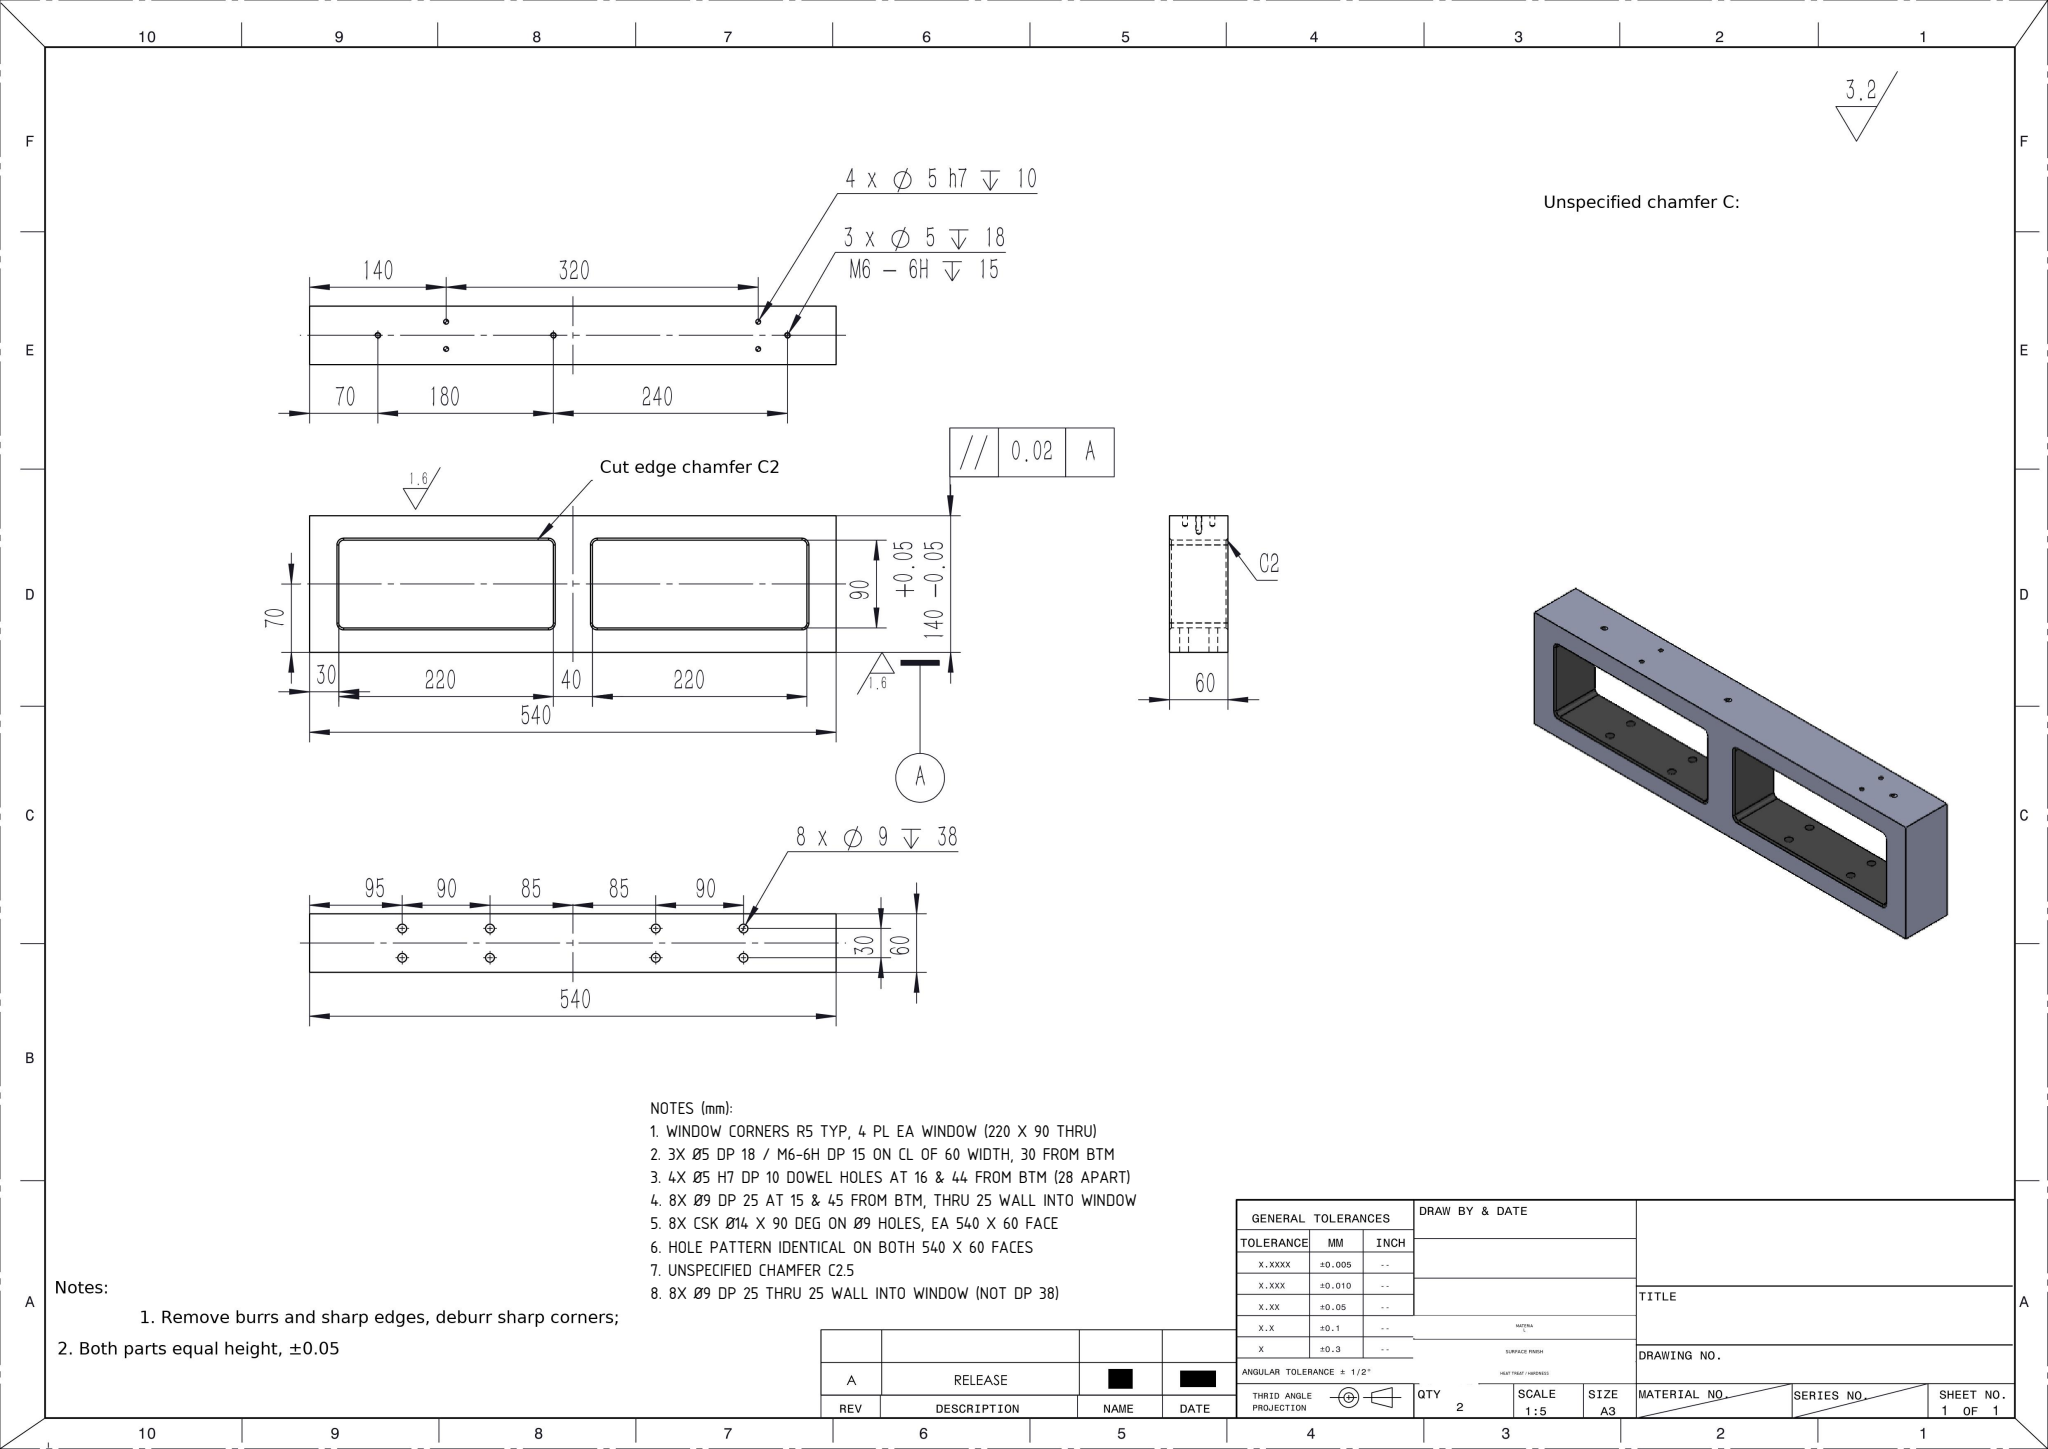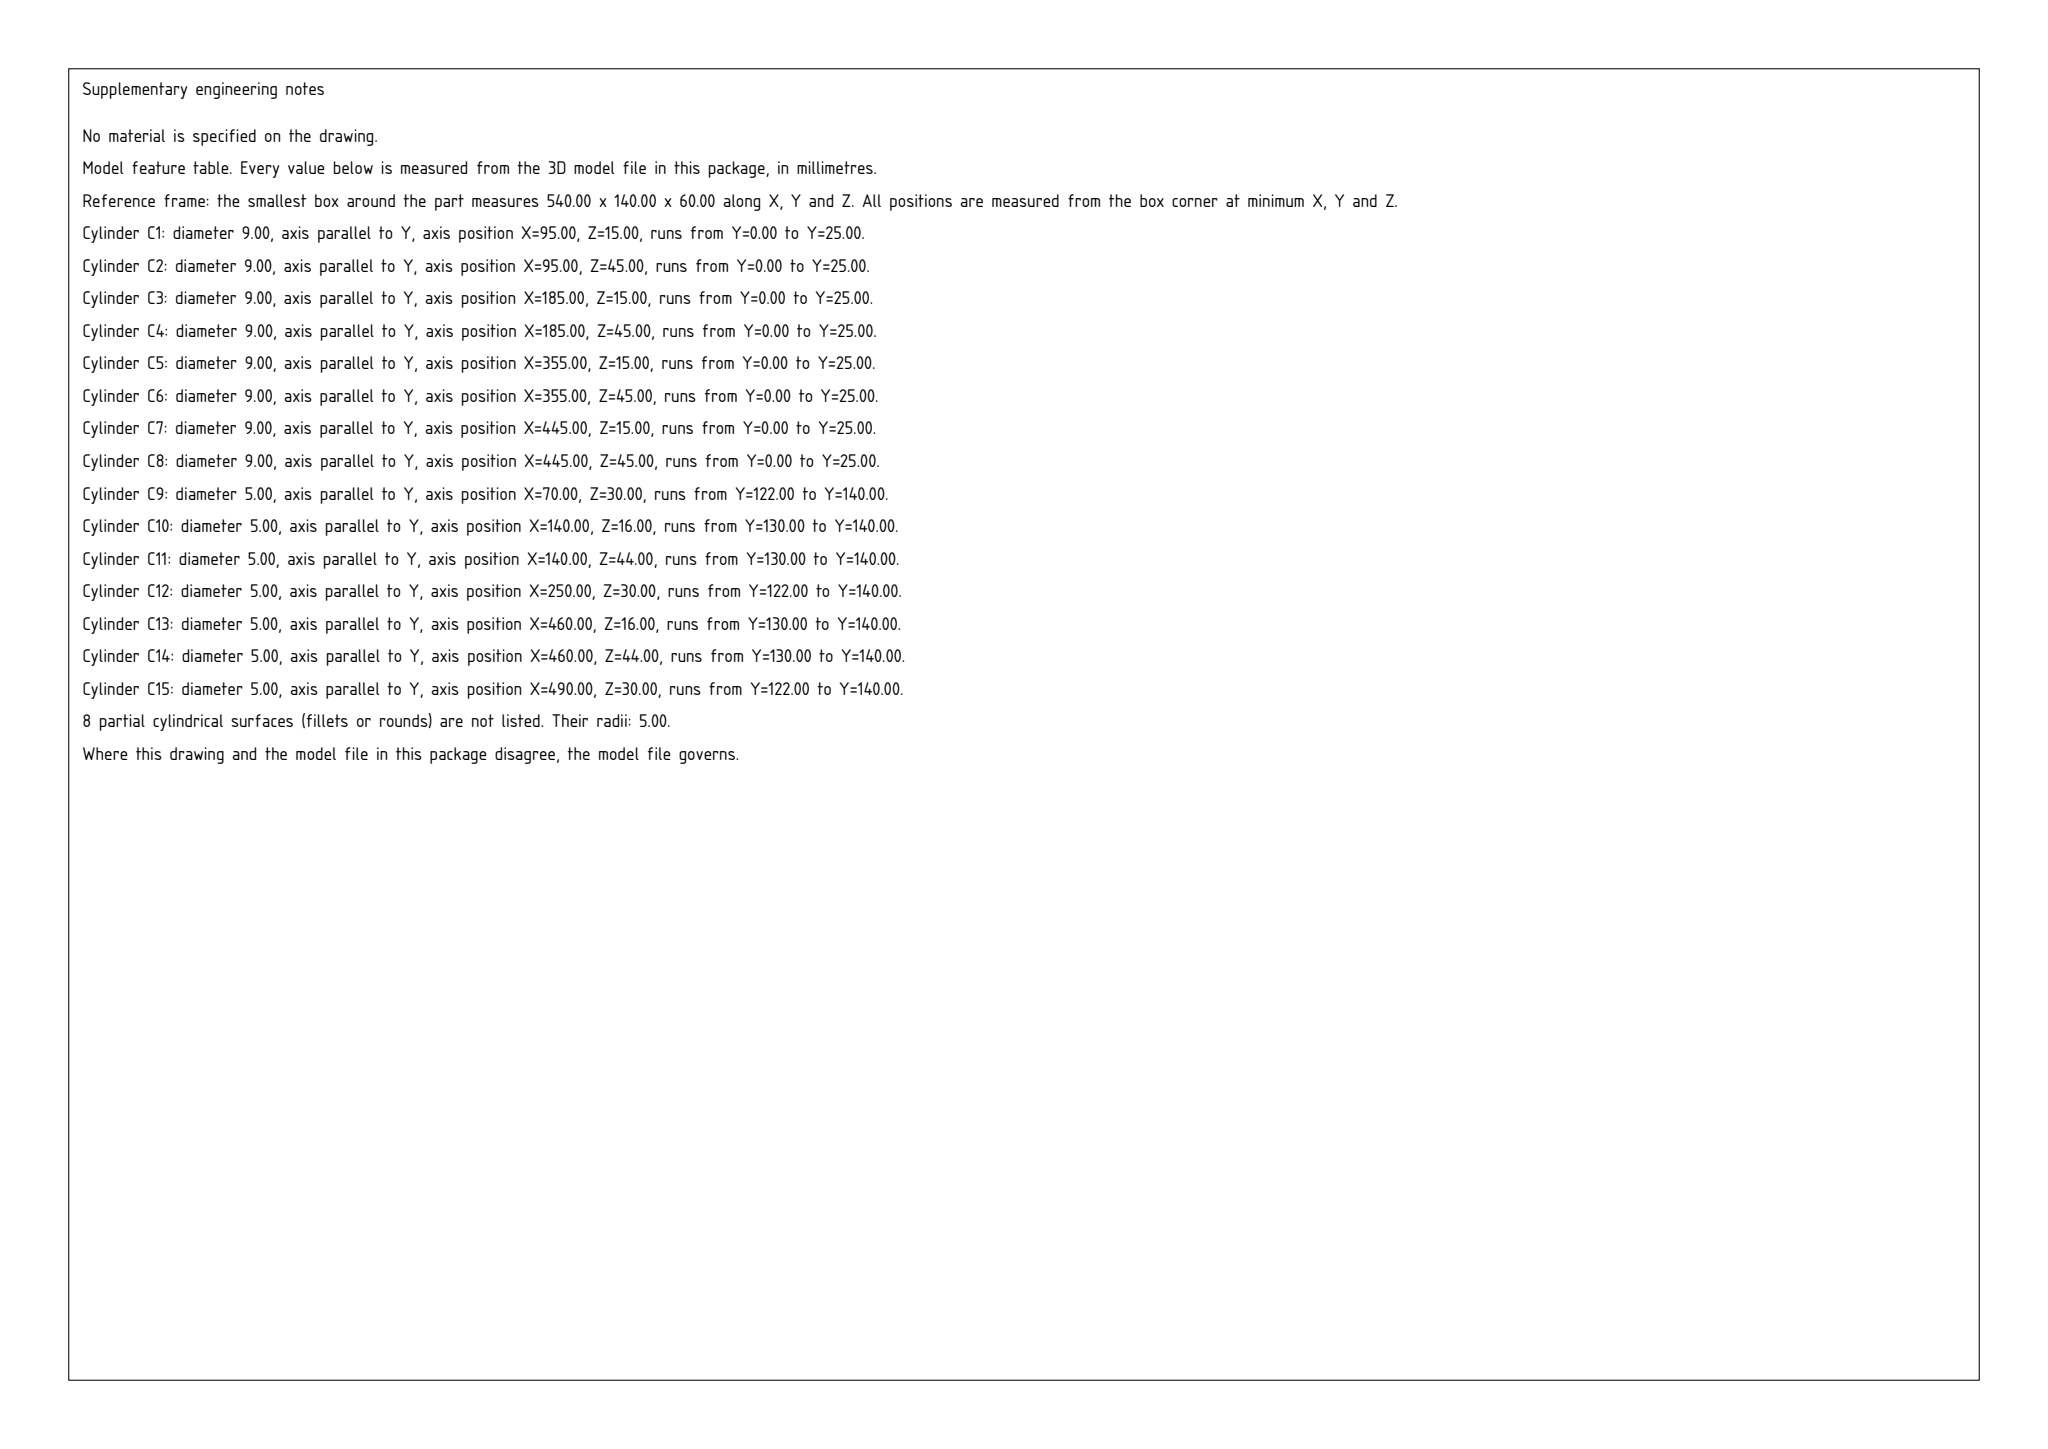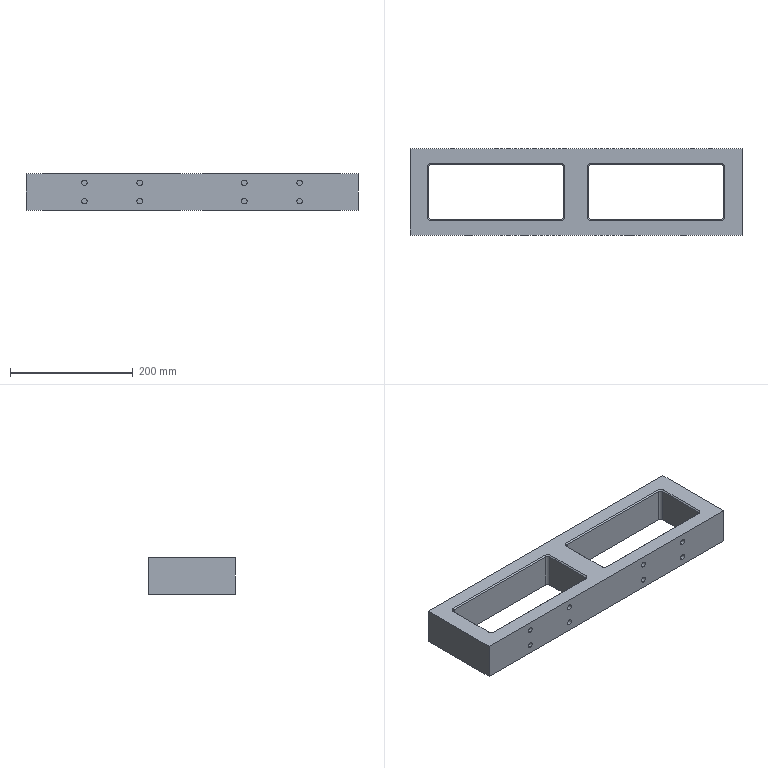Part | SolidWorks | mm | 1 solid | 98 faces | box 540 x 140 x 60 mm | volume 2143012 mm3 | cylinder 38 | cone 30 | plane 30 | commonest cylinder face diameters 9 x16 5 x14 10 x8
Drawing notes:
WINDOW CORNERS R5 TYP, 4 PL EA WINDOW (220 X 90 THRU) | from the solid: Ø10 z-axis cyls at (35,30),(35,110),(245,30),(245,110),(295,30),(295,110),(505,30),(505,110) tangent to window planes x=30/250/290/510, y=25/115 -> R5
3X Ø5 DP 18 / M6-6H DP 15 ON CL OF 60 WIDTH, 30 FROM BTM | from the solid: Ø5 y-axis holes L=18 at z=30, x=70, 250, 490
4X Ø5 H7 DP 10 DOWEL HOLES AT 16 & 44 FROM BTM (28 APART) | from the solid: Ø5 y-axis holes L=10 at z=16 and z=44, x=140 & 460
8X Ø9 DP 25 AT 15 & 45 FROM BTM, THRU 25 WALL INTO WINDOW | from the solid: Ø9 y-axis holes L=25 from y=0/y=140 to window walls y=25/y=115, x=95,185,355,445, z=15 & 45
8X CSK Ø14 X 90 DEG ON Ø9 HOLES, EA 540 X 60 FACE | from the solid: cones [90.0, 14.0] count 16 = 8 holes x 2 faces
HOLE PATTERN IDENTICAL ON BOTH 540 X 60 FACES | from the solid: all Ø5 and Ø9 cylinder entries count=2; cones [118,5] count 14 = 7 holes x 2 faces
UNSPECIFIED CHAMFER C2.5 | from the solid: cones 90 deg incl, ref dia 14 on dia 9 holes -> 2.5 radial chamfer
8X Ø9 DP 25 THRU 25 WALL INTO WINDOW (NOT DP 38) | from the solid: cylinders dia 9, axis y, length 25.0 (8 locations x2 walls)
build123d program:
from build123d import *

# Parameters (mm, degrees)
SKETCH1_W                     = 540
SKETCH1_H                     = 140
BOSS_EXTRUDE1_DEPTH           = 30
M6_TAPPED_HOLE1_D             = 5
M6_TAPPED_HOLE1_DEPTH         = 18
M6_TAPPED_HOLE1_TIP           = 1.502
SIZE_MM_DOWEL_PIN_HOLE1_D     = 5
SIZE_MM_DOWEL_PIN_HOLE1_DEPTH = 10
SIZE_MM_DOWEL_PIN_HOLE1_TIP   = 1.502
SKETCH14_W                    = 220
SKETCH14_H                    = 90
CUT_EXTRUDE1_DEPTH            = 286.307
FILLET1_R                     = 5
M8_CLEARANCE_HOLE1_D          = 9
M8_CLEARANCE_HOLE1_DEPTH      = 38
M8_CLEARANCE_HOLE1_TIP        = 2.704
CHAMFER1_SIZE                 = 2


with BuildPart() as part:
    # Sketch1 → Boss-Extrude1 (new, symmetric)
    with BuildSketch(Plane.XY):
        Rectangle(SKETCH1_W, SKETCH1_H)
    extrude(amount=BOSS_EXTRUDE1_DEPTH, both=True)

    # M6 Tapped Hole1
    with Locations(Plane(origin=(0, 70, 0), x_dir=(-1, 0, 0), z_dir=(0, 1, 0))):
        with Locations((-220, 0), (20, 0), (200, 0)):
            Hole(M6_TAPPED_HOLE1_D / 2, depth=M6_TAPPED_HOLE1_DEPTH)
            with Locations((0, 0, -(M6_TAPPED_HOLE1_DEPTH + M6_TAPPED_HOLE1_TIP / 2))):  # 118° drill point
                Cone(0, M6_TAPPED_HOLE1_D / 2, M6_TAPPED_HOLE1_TIP, mode=Mode.SUBTRACT)

    # Size mm Dowel Pin Hole1
    with Locations(Plane(origin=(0, 70, 0), x_dir=(-1, 0, 0), z_dir=(0, 1, 0))):
        with Locations((-190, -14), (130, -14), (130, 14), (-190, 14)):
            Hole(SIZE_MM_DOWEL_PIN_HOLE1_D / 2, depth=SIZE_MM_DOWEL_PIN_HOLE1_DEPTH)
            with Locations((0, 0, -(SIZE_MM_DOWEL_PIN_HOLE1_DEPTH + SIZE_MM_DOWEL_PIN_HOLE1_TIP / 2))):  # 118° drill point
                Cone(0, SIZE_MM_DOWEL_PIN_HOLE1_D / 2, SIZE_MM_DOWEL_PIN_HOLE1_TIP, mode=Mode.SUBTRACT)

    # Sketch14 → Cut-Extrude1 (cut, through all)
    with BuildSketch(Plane(origin=(0, 0, -30), x_dir=(-1, 0, 0), z_dir=(0, 0, -1))):
        with Locations((-130, 0)):
            Rectangle(SKETCH14_W, SKETCH14_H)
        with Locations((130, 0)):
            Rectangle(SKETCH14_W, SKETCH14_H)
    extrude(amount=-CUT_EXTRUDE1_DEPTH, mode=Mode.SUBTRACT)

    # Fillet1
    fillet1_edges = [part.edges().sort_by_distance(p)[0] for p in [
        (-20, -45, 0),
        (-20, 45, 0),
        (-240, 45, 0),
        (-240, -45, 0),
        (240, 45, 0),
        (20, 45, 0),
        (20, -45, 0),
        (240, -45, 0),
    ]]
    fillet(fillet1_edges, radius=FILLET1_R)

    # M8 Clearance Hole1
    with Locations(Plane(origin=(0, -70, 0), x_dir=(-1, 0, 0), z_dir=(0, -1, 0))):
        with Locations((175, -15), (85, -15), (85, 15), (175, 15), (-175, 15), (-85, 15), (-85, -15), (-175, -15)):
            Hole(M8_CLEARANCE_HOLE1_D / 2, depth=M8_CLEARANCE_HOLE1_DEPTH)
            with Locations((0, 0, -(M8_CLEARANCE_HOLE1_DEPTH + M8_CLEARANCE_HOLE1_TIP / 2))):  # 118° drill point
                Cone(0, M8_CLEARANCE_HOLE1_D / 2, M8_CLEARANCE_HOLE1_TIP, mode=Mode.SUBTRACT)

    # Chamfer1
    chamfer1_edges = [part.edges().sort_by_distance(p)[0] for p in [
        (240, 0, -30),
        (240, 0, 30),
        (130, 45, -30),
        (130, 45, 30),
        (20, 0, -30),
        (20, 0, 30),
        (130, -45, -30),
        (130, -45, 30),
        (-240, 0, -30),
        (-240, 0, 30),
        (-130, -45, -30),
        (-130, -45, 30),
        (-20, 0, -30),
        (-20, 0, 30),
        (-130, 45, -30),
        (-130, 45, 30),
        (238.536, 43.536, -30),
        (238.536, 43.536, 30),
        (21.464, 43.536, -30),
        (21.464, 43.536, 30),
        (21.464, -43.536, -30),
        (21.464, -43.536, 30),
        (238.536, -43.536, -30),
        (238.536, -43.536, 30),
        (-238.536, -43.536, -30),
        (-238.536, -43.536, 30),
        (-21.464, -43.536, -30),
        (-21.464, -43.536, 30),
        (-21.464, 43.536, -30),
        (-21.464, 43.536, 30),
        (-238.536, 43.536, -30),
        (-238.536, 43.536, 30),
    ]]
    chamfer(chamfer1_edges, length=CHAMFER1_SIZE)


solid = part.part